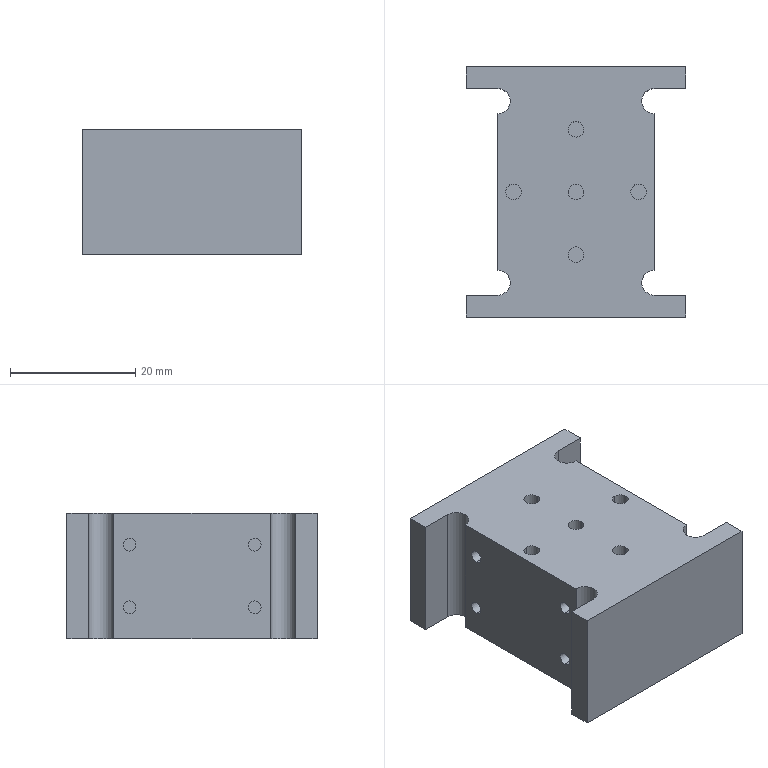CAM job | Mastercam | mm | 10 operations | part box 35 x 40 x 20
1. Facing | 24 - 63 平铣刀
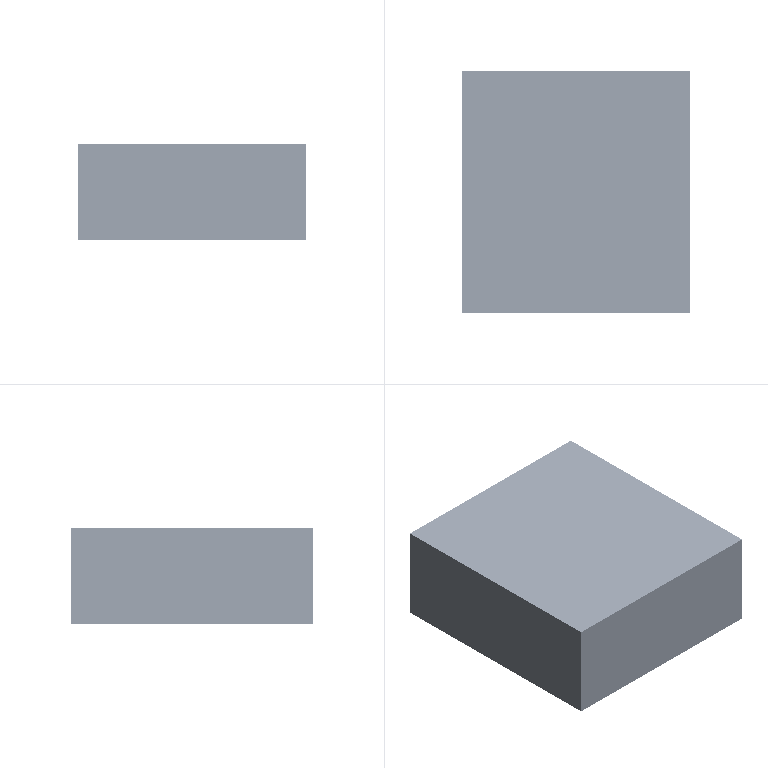2. 2D High Speed (2D Dynamic Mill) | 12 - 12 平铣刀
3. Contour (Remachining) | 4 - 4 平铣刀
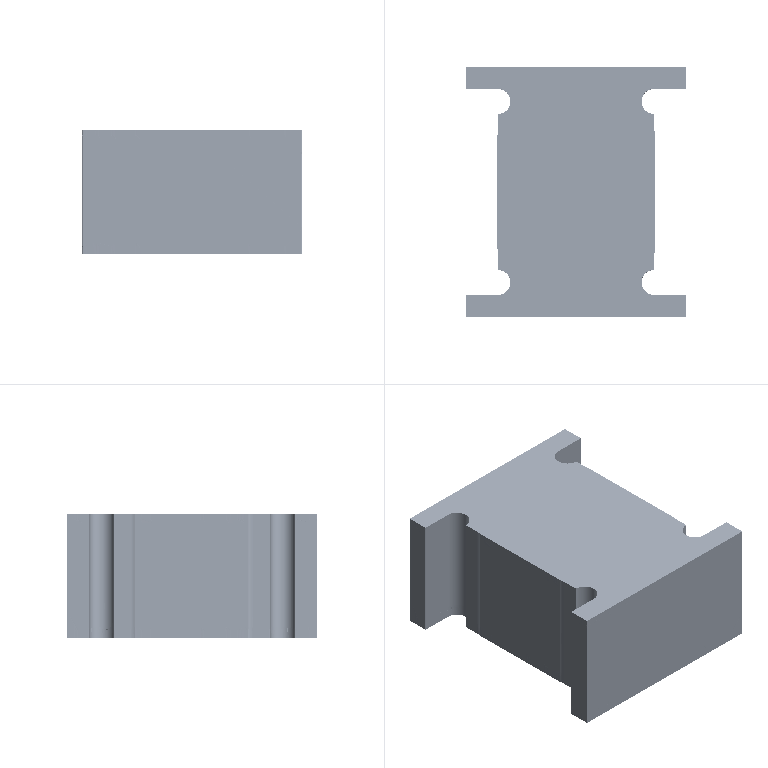4. Contour (2D) | 4 - 4 平铣刀
5. Contour (2D) | 4 - 4 平铣刀
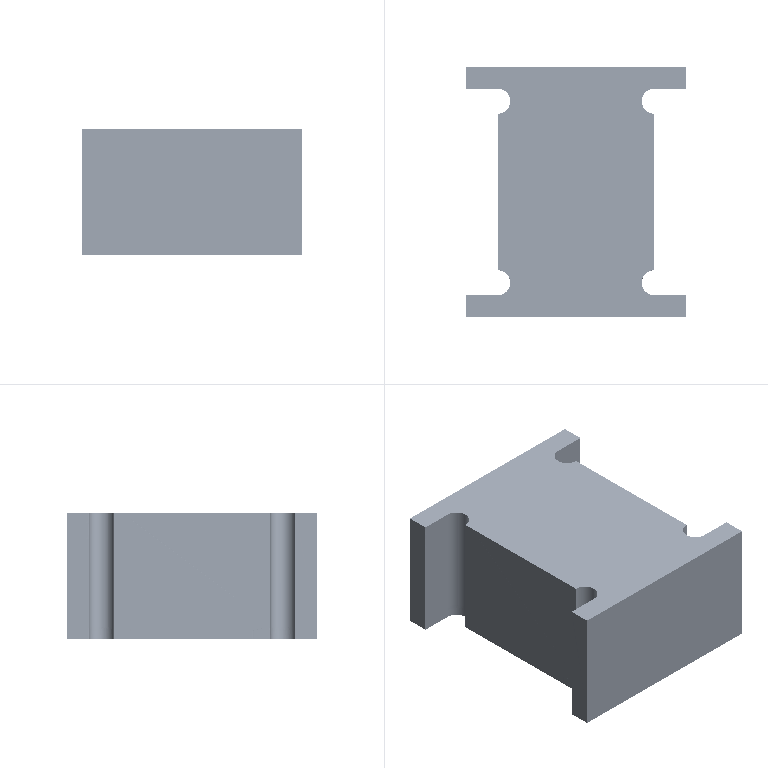6. Drill/Counterbore | 7 - 4 倒角刀
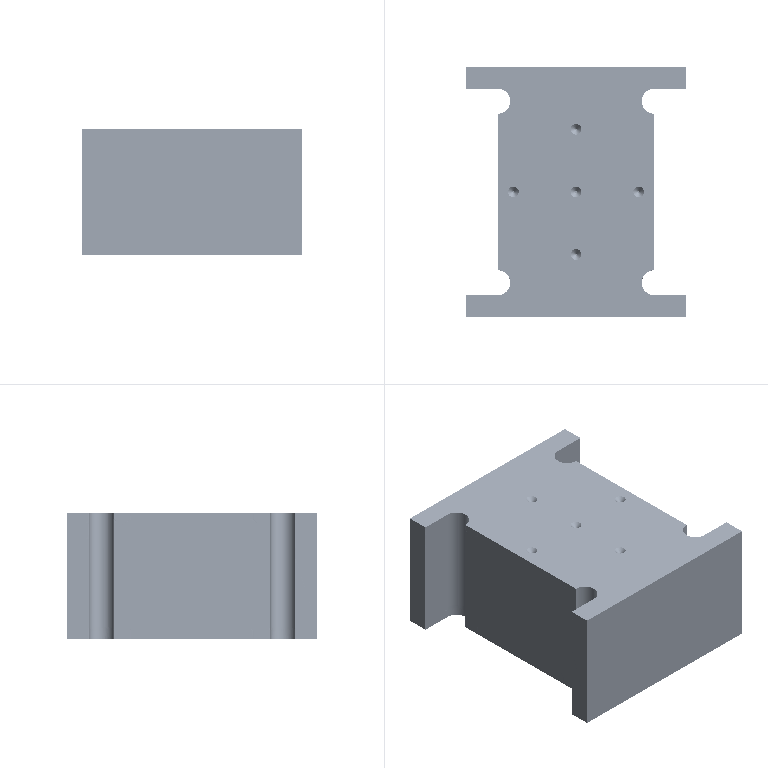7. Contour (2D chamfer) | 7 - 4 倒角刀
8. Facing | 24 - 63 平铣刀
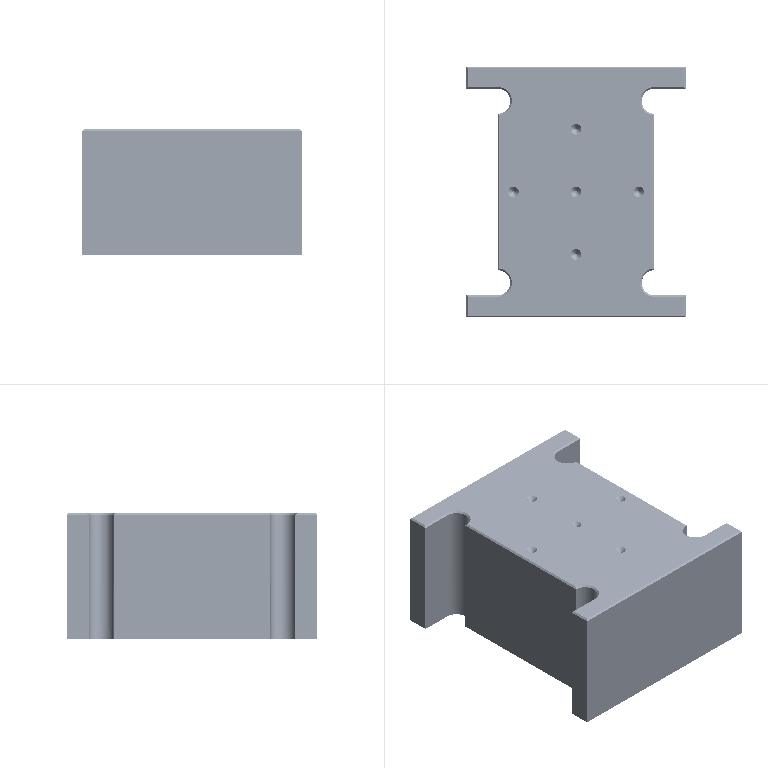9. Contour (2D chamfer) | 7 - 4 倒角刀
10. Drill/Counterbore | 7 - 4 倒角刀